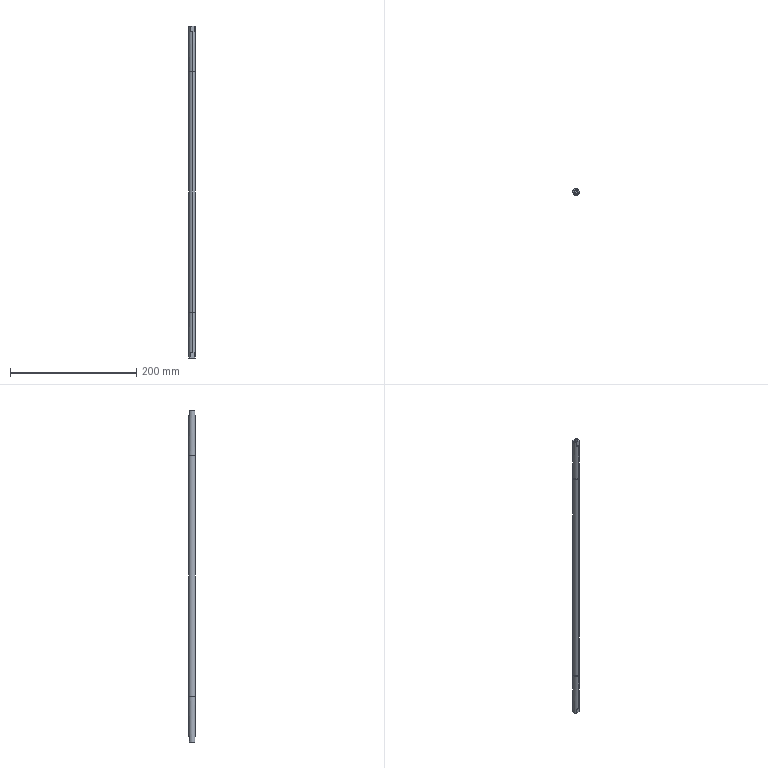Component | SolidWorks | Roller1-1-1_RollerAxis1-1 | 1 solid | 36 faces | box 10 x 10 x 525 mm | volume 40281 mm3 | cylinder 14 | plane 14 | cone 8 | commonest cylinder face diameters 10 x6 5 x4 9.65 x4
build123d program:
from build123d import *

# Parameters (mm, degrees)
CUT_EXTRUDE1_DEPTH           = 8
CUT_EXTRUDE2_DEPTH           = 8
CUT_EXTRUDE3_START           = -8
CUT_EXTRUDE3_DEPTH           = 8
CUT_EXTRUDE4_START           = -8
CUT_EXTRUDE4_DEPTH           = 8
F_5_0_5_DIAMETER_HOLE1_D     = 5
F_5_0_5_DIAMETER_HOLE1_DEPTH = 20
F_5_0_5_DIAMETER_HOLE1_TIP   = 1.502
F_5_0_5_DIAMETER_HOLE2_D     = 5
F_5_0_5_DIAMETER_HOLE2_DEPTH = 20
F_5_0_5_DIAMETER_HOLE2_TIP   = 1.502
CHAMFER1_SIZE                = 0.525


with BuildPart() as part:
    # Sketch1 → Revolve1 (revolve)
    with BuildSketch(Plane(origin=(0, 0, 0), x_dir=(-1, 0, 0), z_dir=(0, 0, -1)), mode=Mode.PRIVATE) as revolve1_sk:
        Polygon((-262.5, 5), (-262.5, 0), (262.5, 0), (262.5, 5), (191.1, 5), (191.1, 4.825), (190, 4.825), (190, 5), (-190, 5), (-190, 4.825), (-191.1, 4.825), (-191.1, 5), align=None)
    revolve(revolve1_sk.sketch.rotate(Axis((262.5, 0, 0), (-1, 0, 0)), 270), axis=Axis((262.5, 0, 0), (-1, 0, 0)))

    # Sketch2 → Cut-Extrude1 (cut)
    with BuildSketch(Plane(origin=(262.5, 0, 0), x_dir=(0, 0, -1), z_dir=(1, 0, 0))):
        with BuildLine():
            Line((4, 3), (4, -3))
            ThreePointArc((4, -3), (5, 0), (4, 3))
        make_face()
    extrude(amount=-CUT_EXTRUDE1_DEPTH, mode=Mode.SUBTRACT)

    # Sketch3 → Cut-Extrude2 (cut)
    with BuildSketch(Plane(origin=(262.5, 0, 0), x_dir=(0, 0, -1), z_dir=(1, 0, 0))):
        with BuildLine():
            Line((-4, -3), (-4, 3))
            ThreePointArc((-4, 3), (-5, 0), (-4, -3))
        make_face()
    extrude(amount=-CUT_EXTRUDE2_DEPTH, mode=Mode.SUBTRACT)

    # Sketch4 → Cut-Extrude3 (cut)
    with BuildSketch(Plane.ZY.offset(262.5).offset(CUT_EXTRUDE3_START)):
        with BuildLine():
            Line((-4, -3), (-4, 3))
            ThreePointArc((-4, 3), (-5, 0), (-4, -3))
        make_face()
    extrude(amount=CUT_EXTRUDE3_DEPTH, mode=Mode.SUBTRACT)

    # Sketch5 → Cut-Extrude4 (cut)
    with BuildSketch(Plane.ZY.offset(262.5).offset(CUT_EXTRUDE4_START)):
        with BuildLine():
            Line((4, 3), (4, -3))
            ThreePointArc((4, -3), (5, 0), (4, 3))
        make_face()
    extrude(amount=CUT_EXTRUDE4_DEPTH, mode=Mode.SUBTRACT)

    # 5.0 _5_ Diameter Hole1
    with Locations(Plane.ZY.offset(262.5)):
        with Locations((0, 0)):
            Hole(F_5_0_5_DIAMETER_HOLE1_D / 2, depth=F_5_0_5_DIAMETER_HOLE1_DEPTH)
            with Locations((0, 0, -(F_5_0_5_DIAMETER_HOLE1_DEPTH + F_5_0_5_DIAMETER_HOLE1_TIP / 2))):  # 118° drill point
                Cone(0, F_5_0_5_DIAMETER_HOLE1_D / 2, F_5_0_5_DIAMETER_HOLE1_TIP, mode=Mode.SUBTRACT)

    # 5.0 _5_ Diameter Hole2
    with Locations(Plane(origin=(262.5, 0, 0), x_dir=(0, 0, -1), z_dir=(1, 0, 0))):
        with Locations((0, 0)):
            Hole(F_5_0_5_DIAMETER_HOLE2_D / 2, depth=F_5_0_5_DIAMETER_HOLE2_DEPTH)
            with Locations((0, 0, -(F_5_0_5_DIAMETER_HOLE2_DEPTH + F_5_0_5_DIAMETER_HOLE2_TIP / 2))):  # 118° drill point
                Cone(0, F_5_0_5_DIAMETER_HOLE2_D / 2, F_5_0_5_DIAMETER_HOLE2_TIP, mode=Mode.SUBTRACT)

    # Chamfer1
    chamfer1_edges = [part.edges().sort_by_distance(p)[0] for p in [
        (-262.5, 0, 2.5),
        (262.5, 0, -2.5),
    ]]
    chamfer(chamfer1_edges, length=CHAMFER1_SIZE)


solid = part.part

# Placed as in the assembly
solid = solid.moved(Location((-44.993, 283.892, 0), (90, 5.533, 90)))
STEP:
#1=COLOUR_RGB('',0.7922,0.8196,0.9333);
#2=FILL_AREA_STYLE_COLOUR('',#1);
#3=FILL_AREA_STYLE('',(#2));
#4=SURFACE_STYLE_FILL_AREA(#3);
#5=SURFACE_SIDE_STYLE('',(#4));
#6=SURFACE_STYLE_USAGE(.BOTH.,#5);
#7=PRESENTATION_STYLE_ASSIGNMENT((#6));
#8=CARTESIAN_POINT('',(-1.762,11.079,-10.314));
#9=VERTEX_POINT('',#8);
#10=CARTESIAN_POINT('',(-1.781,11.275,-10.314));
#11=VERTEX_POINT('',#10);
#12=CARTESIAN_POINT('',(-1.771,11.177,-10.314));
#13=DIRECTION('',(-0.,0.,-1.));
#14=DIRECTION('',(-0.09642,0.9953,0.));
#15=AXIS2_PLACEMENT_3D('',#12,#13,#14);
#16=CIRCLE('',#15,0.09843);
#17=EDGE_CURVE('',#9,#11,#16,.T.);
#18=ORIENTED_EDGE('',*,*,#17,.F.);
#19=CARTESIAN_POINT('',(-1.76,11.058,-10.335));
#20=VERTEX_POINT('',#19);
#21=CARTESIAN_POINT('',(-1.762,11.079,-10.314));
#22=DIRECTION('',(0.06818,-0.7038,-0.7071));
#23=VECTOR('',#22,39.37);
#24=LINE('',#21,#23);
#25=EDGE_CURVE('',#9,#20,#24,.T.);
#26=ORIENTED_EDGE('',*,*,#25,.T.);
#27=CARTESIAN_POINT('',(-1.783,11.295,-10.335));
#28=VERTEX_POINT('',#27);
#29=CARTESIAN_POINT('',(-1.771,11.177,-10.335));
#30=DIRECTION('',(0.,-0.,1.));
#31=DIRECTION('',(-0.09642,0.9953,0.));
#32=AXIS2_PLACEMENT_3D('',#29,#30,#31);
#33=CIRCLE('',#32,0.1191);
#34=EDGE_CURVE('',#28,#20,#33,.T.);
#35=ORIENTED_EDGE('',*,*,#34,.F.);
#36=CARTESIAN_POINT('',(-1.781,11.275,-10.314));
#37=DIRECTION('',(-0.06818,0.7038,-0.7071));
#38=VECTOR('',#37,39.37);
#39=LINE('',#36,#38);
#40=EDGE_CURVE('',#11,#28,#39,.T.);
#41=ORIENTED_EDGE('',*,*,#40,.F.);
#42=EDGE_LOOP('',(#18,#26,#35,#41));
#43=FACE_OUTER_BOUND('',#42,.T.);
#44=CARTESIAN_POINT('',(-1.771,11.177,-10.314));
#45=DIRECTION('',(-0.,0.,-1.));
#46=DIRECTION('',(-0.09642,0.9953,0.));
#47=AXIS2_PLACEMENT_3D('',#44,#45,#46);
#48=CONICAL_SURFACE('',#47,0.09843,0.7854);
#49=ADVANCED_FACE('',(#43),#48,.F.);
#50=CARTESIAN_POINT('',(-1.781,11.275,10.314));
#51=VERTEX_POINT('',#50);
#52=CARTESIAN_POINT('',(-1.762,11.079,10.314));
#53=VERTEX_POINT('',#52);
#54=CARTESIAN_POINT('',(-1.771,11.177,10.314));
#55=DIRECTION('',(0.,-0.,1.));
#56=DIRECTION('',(0.09642,-0.9953,0.));
#57=AXIS2_PLACEMENT_3D('',#54,#55,#56);
#58=CIRCLE('',#57,0.09843);
#59=EDGE_CURVE('',#51,#53,#58,.T.);
#60=ORIENTED_EDGE('',*,*,#59,.F.);
#61=CARTESIAN_POINT('',(-1.783,11.295,10.335));
#62=VERTEX_POINT('',#61);
#63=CARTESIAN_POINT('',(-1.781,11.275,10.314));
#64=DIRECTION('',(-0.06818,0.7038,0.7071));
#65=VECTOR('',#64,39.37);
#66=LINE('',#63,#65);
#67=EDGE_CURVE('',#51,#62,#66,.T.);
#68=ORIENTED_EDGE('',*,*,#67,.T.);
#69=CARTESIAN_POINT('',(-1.76,11.058,10.335));
#70=VERTEX_POINT('',#69);
#71=CARTESIAN_POINT('',(-1.771,11.177,10.335));
#72=DIRECTION('',(-0.,0.,-1.));
#73=DIRECTION('',(0.09642,-0.9953,0.));
#74=AXIS2_PLACEMENT_3D('',#71,#72,#73);
#75=CIRCLE('',#74,0.1191);
#76=EDGE_CURVE('',#70,#62,#75,.T.);
#77=ORIENTED_EDGE('',*,*,#76,.F.);
#78=CARTESIAN_POINT('',(-1.762,11.079,10.314));
#79=DIRECTION('',(0.06818,-0.7038,0.7071));
#80=VECTOR('',#79,39.37);
#81=LINE('',#78,#80);
#82=EDGE_CURVE('',#53,#70,#81,.T.);
#83=ORIENTED_EDGE('',*,*,#82,.F.);
#84=EDGE_LOOP('',(#60,#68,#77,#83));
#85=FACE_OUTER_BOUND('',#84,.T.);
#86=CARTESIAN_POINT('',(-1.771,11.177,10.314));
#87=DIRECTION('',(0.,-0.,1.));
#88=DIRECTION('',(0.09642,-0.9953,0.));
#89=AXIS2_PLACEMENT_3D('',#86,#87,#88);
#90=CONICAL_SURFACE('',#89,0.09843,0.7854);
#91=ADVANCED_FACE('',(#85),#90,.F.);
#92=CARTESIAN_POINT('',(-1.762,11.079,-9.547));
#93=VERTEX_POINT('',#92);
#94=CARTESIAN_POINT('',(-1.781,11.275,-9.547));
#95=VERTEX_POINT('',#94);
#96=CARTESIAN_POINT('',(-1.771,11.177,-9.547));
#97=DIRECTION('',(-0.,0.,-1.));
#98=DIRECTION('',(-0.09642,0.9953,0.));
#99=AXIS2_PLACEMENT_3D('',#96,#97,#98);
#100=CIRCLE('',#99,0.09843);
#101=EDGE_CURVE('',#93,#95,#100,.T.);
#102=ORIENTED_EDGE('',*,*,#101,.F.);
#103=CARTESIAN_POINT('',(-1.762,11.079,-10.335));
#104=DIRECTION('',(-0.,0.,-1.));
#105=VECTOR('',#104,39.37);
#106=LINE('',#103,#105);
#107=EDGE_CURVE('',#93,#9,#106,.T.);
#108=ORIENTED_EDGE('',*,*,#107,.T.);
#109=ORIENTED_EDGE('',*,*,#17,.T.);
#110=CARTESIAN_POINT('',(-1.781,11.275,-10.335));
#111=DIRECTION('',(-0.,0.,-1.));
#112=VECTOR('',#111,39.37);
#113=LINE('',#110,#112);
#114=EDGE_CURVE('',#95,#11,#113,.T.);
#115=ORIENTED_EDGE('',*,*,#114,.F.);
#116=EDGE_LOOP('',(#102,#108,#109,#115));
#117=FACE_OUTER_BOUND('',#116,.T.);
#118=CARTESIAN_POINT('',(-1.771,11.177,-10.335));
#119=DIRECTION('',(-0.,0.,-1.));
#120=DIRECTION('',(-0.09642,0.9953,0.));
#121=AXIS2_PLACEMENT_3D('',#118,#119,#120);
#122=CYLINDRICAL_SURFACE('',#121,0.09843);
#123=ADVANCED_FACE('',(#117),#122,.F.);
#124=CARTESIAN_POINT('',(-1.771,11.177,-9.488));
#125=VERTEX_POINT('',#124);
#126=CARTESIAN_POINT('',(-1.781,11.275,-9.547));
#127=DIRECTION('',(-0.08265,0.8532,-0.515));
#128=VECTOR('',#127,39.37);
#129=LINE('',#126,#128);
#130=EDGE_CURVE('',#125,#95,#129,.T.);
#131=ORIENTED_EDGE('',*,*,#130,.F.);
#132=CARTESIAN_POINT('',(-1.762,11.079,-9.547));
#133=DIRECTION('',(0.08265,-0.8532,-0.515));
#134=VECTOR('',#133,39.37);
#135=LINE('',#132,#134);
#136=EDGE_CURVE('',#125,#93,#135,.T.);
#137=ORIENTED_EDGE('',*,*,#136,.T.);
#138=ORIENTED_EDGE('',*,*,#101,.T.);
#139=EDGE_LOOP('',(#131,#137,#138));
#140=FACE_OUTER_BOUND('',#139,.T.);
#141=CARTESIAN_POINT('',(-1.771,11.177,-9.547));
#142=DIRECTION('',(-0.,0.,-1.));
#143=DIRECTION('',(-0.09642,0.9953,0.));
#144=AXIS2_PLACEMENT_3D('',#141,#142,#143);
#145=CONICAL_SURFACE('',#144,0.09843,1.03);
#146=ADVANCED_FACE('',(#140),#145,.F.);
#147=CARTESIAN_POINT('',(-1.781,11.275,9.547));
#148=VERTEX_POINT('',#147);
#149=CARTESIAN_POINT('',(-1.762,11.079,9.547));
#150=VERTEX_POINT('',#149);
#151=CARTESIAN_POINT('',(-1.771,11.177,9.547));
#152=DIRECTION('',(0.,-0.,1.));
#153=DIRECTION('',(0.09642,-0.9953,0.));
#154=AXIS2_PLACEMENT_3D('',#151,#152,#153);
#155=CIRCLE('',#154,0.09843);
#156=EDGE_CURVE('',#148,#150,#155,.T.);
#157=ORIENTED_EDGE('',*,*,#156,.F.);
#158=CARTESIAN_POINT('',(-1.781,11.275,10.335));
#159=DIRECTION('',(0.,-0.,1.));
#160=VECTOR('',#159,39.37);
#161=LINE('',#158,#160);
#162=EDGE_CURVE('',#148,#51,#161,.T.);
#163=ORIENTED_EDGE('',*,*,#162,.T.);
#164=ORIENTED_EDGE('',*,*,#59,.T.);
#165=CARTESIAN_POINT('',(-1.762,11.079,10.335));
#166=DIRECTION('',(0.,-0.,1.));
#167=VECTOR('',#166,39.37);
#168=LINE('',#165,#167);
#169=EDGE_CURVE('',#150,#53,#168,.T.);
#170=ORIENTED_EDGE('',*,*,#169,.F.);
#171=EDGE_LOOP('',(#157,#163,#164,#170));
#172=FACE_OUTER_BOUND('',#171,.T.);
#173=CARTESIAN_POINT('',(-1.771,11.177,10.335));
#174=DIRECTION('',(0.,-0.,1.));
#175=DIRECTION('',(0.09642,-0.9953,0.));
#176=AXIS2_PLACEMENT_3D('',#173,#174,#175);
#177=CYLINDRICAL_SURFACE('',#176,0.09843);
#178=ADVANCED_FACE('',(#172),#177,.F.);
#179=CARTESIAN_POINT('',(-1.771,11.177,9.488));
#180=VERTEX_POINT('',#179);
#181=CARTESIAN_POINT('',(-1.762,11.079,9.547));
#182=DIRECTION('',(0.08265,-0.8532,0.515));
#183=VECTOR('',#182,39.37);
#184=LINE('',#181,#183);
#185=EDGE_CURVE('',#180,#150,#184,.T.);
#186=ORIENTED_EDGE('',*,*,#185,.F.);
#187=CARTESIAN_POINT('',(-1.781,11.275,9.547));
#188=DIRECTION('',(-0.08265,0.8532,0.515));
#189=VECTOR('',#188,39.37);
#190=LINE('',#187,#189);
#191=EDGE_CURVE('',#180,#148,#190,.T.);
#192=ORIENTED_EDGE('',*,*,#191,.T.);
#193=ORIENTED_EDGE('',*,*,#156,.T.);
#194=EDGE_LOOP('',(#186,#192,#193));
#195=FACE_OUTER_BOUND('',#194,.T.);
#196=CARTESIAN_POINT('',(-1.771,11.177,9.547));
#197=DIRECTION('',(0.,-0.,1.));
#198=DIRECTION('',(0.09642,-0.9953,0.));
#199=AXIS2_PLACEMENT_3D('',#196,#197,#198);
#200=CONICAL_SURFACE('',#199,0.09843,1.03);
#201=ADVANCED_FACE('',(#195),#200,.F.);
#202=CARTESIAN_POINT('',(-1.753,10.988,-7.524));
#203=VERTEX_POINT('',#202);
#204=CARTESIAN_POINT('',(-1.79,11.366,-7.524));
#205=VERTEX_POINT('',#204);
#206=CARTESIAN_POINT('',(-1.771,11.177,-7.524));
#207=DIRECTION('',(0.,-0.,1.));
#208=DIRECTION('',(0.09642,-0.9953,0.));
#209=AXIS2_PLACEMENT_3D('',#206,#207,#208);
#210=CIRCLE('',#209,0.19);
#211=EDGE_CURVE('',#203,#205,#210,.T.);
#212=ORIENTED_EDGE('',*,*,#211,.T.);
#213=CARTESIAN_POINT('',(-1.79,11.366,-7.48));
#214=VERTEX_POINT('',#213);
#215=CARTESIAN_POINT('',(-1.79,11.366,-10.335));
#216=DIRECTION('',(0.,-0.,1.));
#217=VECTOR('',#216,39.37);
#218=LINE('',#215,#217);
#219=EDGE_CURVE('',#205,#214,#218,.T.);
#220=ORIENTED_EDGE('',*,*,#219,.T.);
#221=CARTESIAN_POINT('',(-1.753,10.988,-7.48));
#222=VERTEX_POINT('',#221);
#223=CARTESIAN_POINT('',(-1.771,11.177,-7.48));
#224=DIRECTION('',(0.,-0.,1.));
#225=DIRECTION('',(0.09642,-0.9953,0.));
#226=AXIS2_PLACEMENT_3D('',#223,#224,#225);
#227=CIRCLE('',#226,0.19);
#228=EDGE_CURVE('',#222,#214,#227,.T.);
#229=ORIENTED_EDGE('',*,*,#228,.F.);
#230=CARTESIAN_POINT('',(-1.753,10.988,-10.335));
#231=DIRECTION('',(0.,-0.,1.));
#232=VECTOR('',#231,39.37);
#233=LINE('',#230,#232);
#234=EDGE_CURVE('',#203,#222,#233,.T.);
#235=ORIENTED_EDGE('',*,*,#234,.F.);
#236=EDGE_LOOP('',(#212,#220,#229,#235));
#237=FACE_OUTER_BOUND('',#236,.T.);
#238=CARTESIAN_POINT('',(-1.771,11.177,-10.335));
#239=DIRECTION('',(0.,-0.,1.));
#240=DIRECTION('',(0.09642,-0.9953,0.));
#241=AXIS2_PLACEMENT_3D('',#238,#239,#240);
#242=CYLINDRICAL_SURFACE('',#241,0.19);
#243=ADVANCED_FACE('',(#237),#242,.T.);
#244=CARTESIAN_POINT('',(-1.752,10.981,-7.48));
#245=VERTEX_POINT('',#244);
#246=CARTESIAN_POINT('',(-1.79,11.373,-7.48));
#247=VERTEX_POINT('',#246);
#248=CARTESIAN_POINT('',(-1.771,11.177,-7.48));
#249=DIRECTION('',(0.,-0.,1.));
#250=DIRECTION('',(0.09642,-0.9953,0.));
#251=AXIS2_PLACEMENT_3D('',#248,#249,#250);
#252=CIRCLE('',#251,0.1969);
#253=EDGE_CURVE('',#245,#247,#252,.T.);
#254=ORIENTED_EDGE('',*,*,#253,.T.);
#255=CARTESIAN_POINT('',(-1.79,11.373,7.48));
#256=VERTEX_POINT('',#255);
#257=CARTESIAN_POINT('',(-1.79,11.373,-10.335));
#258=DIRECTION('',(0.,-0.,1.));
#259=VECTOR('',#258,39.37);
#260=LINE('',#257,#259);
#261=EDGE_CURVE('',#247,#256,#260,.T.);
#262=ORIENTED_EDGE('',*,*,#261,.T.);
#263=CARTESIAN_POINT('',(-1.752,10.981,7.48));
#264=VERTEX_POINT('',#263);
#265=CARTESIAN_POINT('',(-1.771,11.177,7.48));
#266=DIRECTION('',(0.,-0.,1.));
#267=DIRECTION('',(0.09642,-0.9953,0.));
#268=AXIS2_PLACEMENT_3D('',#265,#266,#267);
#269=CIRCLE('',#268,0.1969);
#270=EDGE_CURVE('',#264,#256,#269,.T.);
#271=ORIENTED_EDGE('',*,*,#270,.F.);
#272=CARTESIAN_POINT('',(-1.752,10.981,-10.335));
#273=DIRECTION('',(0.,-0.,1.));
#274=VECTOR('',#273,39.37);
#275=LINE('',#272,#274);
#276=EDGE_CURVE('',#245,#264,#275,.T.);
#277=ORIENTED_EDGE('',*,*,#276,.F.);
#278=EDGE_LOOP('',(#254,#262,#271,#277));
#279=FACE_OUTER_BOUND('',#278,.T.);
#280=CARTESIAN_POINT('',(-1.771,11.177,-10.335));
#281=DIRECTION('',(0.,-0.,1.));
#282=DIRECTION('',(0.09642,-0.9953,0.));
#283=AXIS2_PLACEMENT_3D('',#280,#281,#282);
#284=CYLINDRICAL_SURFACE('',#283,0.1969);
#285=ADVANCED_FACE('',(#279),#284,.T.);
#286=CARTESIAN_POINT('',(-1.753,10.988,7.48));
#287=VERTEX_POINT('',#286);
#288=CARTESIAN_POINT('',(-1.79,11.366,7.48));
#289=VERTEX_POINT('',#288);
#290=CARTESIAN_POINT('',(-1.771,11.177,7.48));
#291=DIRECTION('',(0.,-0.,1.));
#292=DIRECTION('',(0.09642,-0.9953,0.));
#293=AXIS2_PLACEMENT_3D('',#290,#291,#292);
#294=CIRCLE('',#293,0.19);
#295=EDGE_CURVE('',#287,#289,#294,.T.);
#296=ORIENTED_EDGE('',*,*,#295,.T.);
#297=CARTESIAN_POINT('',(-1.79,11.366,7.524));
#298=VERTEX_POINT('',#297);
#299=CARTESIAN_POINT('',(-1.79,11.366,-10.335));
#300=DIRECTION('',(0.,-0.,1.));
#301=VECTOR('',#300,39.37);
#302=LINE('',#299,#301);
#303=EDGE_CURVE('',#289,#298,#302,.T.);
#304=ORIENTED_EDGE('',*,*,#303,.T.);
#305=CARTESIAN_POINT('',(-1.753,10.988,7.524));
#306=VERTEX_POINT('',#305);
#307=CARTESIAN_POINT('',(-1.771,11.177,7.524));
#308=DIRECTION('',(0.,-0.,1.));
#309=DIRECTION('',(0.09642,-0.9953,0.));
#310=AXIS2_PLACEMENT_3D('',#307,#308,#309);
#311=CIRCLE('',#310,0.19);
#312=EDGE_CURVE('',#306,#298,#311,.T.);
#313=ORIENTED_EDGE('',*,*,#312,.F.);
#314=CARTESIAN_POINT('',(-1.753,10.988,-10.335));
#315=DIRECTION('',(0.,-0.,1.));
#316=VECTOR('',#315,39.37);
#317=LINE('',#314,#316);
#318=EDGE_CURVE('',#287,#306,#317,.T.);
#319=ORIENTED_EDGE('',*,*,#318,.F.);
#320=EDGE_LOOP('',(#296,#304,#313,#319));
#321=FACE_OUTER_BOUND('',#320,.T.);
#322=CARTESIAN_POINT('',(-1.771,11.177,-10.335));
#323=DIRECTION('',(0.,-0.,1.));
#324=DIRECTION('',(0.09642,-0.9953,0.));
#325=AXIS2_PLACEMENT_3D('',#322,#323,#324);
#326=CYLINDRICAL_SURFACE('',#325,0.19);
#327=ADVANCED_FACE('',(#321),#326,.T.);
#328=CARTESIAN_POINT('',(-1.752,10.981,7.524));
#329=VERTEX_POINT('',#328);
#330=CARTESIAN_POINT('',(-1.79,11.373,7.524));
#331=VERTEX_POINT('',#330);
#332=CARTESIAN_POINT('',(-1.771,11.177,7.524));
#333=DIRECTION('',(0.,-0.,1.));
#334=DIRECTION('',(0.09642,-0.9953,0.));
#335=AXIS2_PLACEMENT_3D('',#332,#333,#334);
#336=CIRCLE('',#335,0.1969);
#337=EDGE_CURVE('',#329,#331,#336,.T.);
#338=ORIENTED_EDGE('',*,*,#337,.T.);
#339=CARTESIAN_POINT('',(-1.79,11.373,10.02));
#340=VERTEX_POINT('',#339);
#341=CARTESIAN_POINT('',(-1.79,11.373,-10.335));
#342=DIRECTION('',(0.,-0.,1.));
#343=VECTOR('',#342,39.37);
#344=LINE('',#341,#343);
#345=EDGE_CURVE('',#331,#340,#344,.T.);
#346=ORIENTED_EDGE('',*,*,#345,.T.);
#347=CARTESIAN_POINT('',(-1.669,11.345,10.02));
#348=VERTEX_POINT('',#347);
#349=CARTESIAN_POINT('',(-1.771,11.177,10.02));
#350=DIRECTION('',(0.,-0.,1.));
#351=DIRECTION('',(0.09642,-0.9953,0.));
#352=AXIS2_PLACEMENT_3D('',#349,#350,#351);
#353=CIRCLE('',#352,0.1969);
#354=EDGE_CURVE('',#348,#340,#353,.T.);
#355=ORIENTED_EDGE('',*,*,#354,.F.);
#356=CARTESIAN_POINT('',(-1.669,11.345,10.335));
#357=VERTEX_POINT('',#356);
#358=CARTESIAN_POINT('',(-1.669,11.345,10.02));
#359=DIRECTION('',(0.,-0.,1.));
#360=VECTOR('',#359,39.37);
#361=LINE('',#358,#360);
#362=EDGE_CURVE('',#348,#357,#361,.T.);
#363=ORIENTED_EDGE('',*,*,#362,.T.);
#364=CARTESIAN_POINT('',(-1.639,11.031,10.335));
#365=VERTEX_POINT('',#364);
#366=CARTESIAN_POINT('',(-1.771,11.177,10.335));
#367=DIRECTION('',(0.,-0.,1.));
#368=DIRECTION('',(0.09642,-0.9953,0.));
#369=AXIS2_PLACEMENT_3D('',#366,#367,#368);
#370=CIRCLE('',#369,0.1969);
#371=EDGE_CURVE('',#365,#357,#370,.T.);
#372=ORIENTED_EDGE('',*,*,#371,.F.);
#373=CARTESIAN_POINT('',(-1.639,11.031,10.02));
#374=VERTEX_POINT('',#373);
#375=CARTESIAN_POINT('',(-1.639,11.031,10.02));
#376=DIRECTION('',(0.,-0.,1.));
#377=VECTOR('',#376,39.37);
#378=LINE('',#375,#377);
#379=EDGE_CURVE('',#374,#365,#378,.T.);
#380=ORIENTED_EDGE('',*,*,#379,.F.);
#381=CARTESIAN_POINT('',(-1.752,10.981,10.02));
#382=VERTEX_POINT('',#381);
#383=CARTESIAN_POINT('',(-1.771,11.177,10.02));
#384=DIRECTION('',(0.,-0.,1.));
#385=DIRECTION('',(0.09642,-0.9953,0.));
#386=AXIS2_PLACEMENT_3D('',#383,#384,#385);
#387=CIRCLE('',#386,0.1969);
#388=EDGE_CURVE('',#382,#374,#387,.T.);
#389=ORIENTED_EDGE('',*,*,#388,.F.);
#390=CARTESIAN_POINT('',(-1.752,10.981,-10.335));
#391=DIRECTION('',(0.,-0.,1.));
#392=VECTOR('',#391,39.37);
#393=LINE('',#390,#392);
#394=EDGE_CURVE('',#329,#382,#393,.T.);
#395=ORIENTED_EDGE('',*,*,#394,.F.);
#396=EDGE_LOOP('',(#338,#346,#355,#363,#372,#380,#389,#395));
#397=FACE_OUTER_BOUND('',#396,.T.);
#398=CARTESIAN_POINT('',(-1.771,11.177,-10.335));
#399=DIRECTION('',(0.,-0.,1.));
#400=DIRECTION('',(0.09642,-0.9953,0.));
#401=AXIS2_PLACEMENT_3D('',#398,#399,#400);
#402=CYLINDRICAL_SURFACE('',#401,0.1969);
#403=ADVANCED_FACE('',(#397),#402,.T.);
#404=CARTESIAN_POINT('',(-1.79,11.373,-10.02));
#405=VERTEX_POINT('',#404);
#406=CARTESIAN_POINT('',(-1.669,11.345,-10.02));
#407=VERTEX_POINT('',#406);
#408=CARTESIAN_POINT('',(-1.771,11.177,-10.02));
#409=DIRECTION('',(-0.,0.,-1.));
#410=DIRECTION('',(-0.09642,0.9953,0.));
#411=AXIS2_PLACEMENT_3D('',#408,#409,#410);
#412=CIRCLE('',#411,0.1969);
#413=EDGE_CURVE('',#405,#407,#412,.T.);
#414=ORIENTED_EDGE('',*,*,#413,.F.);
#415=CARTESIAN_POINT('',(-1.79,11.373,-7.524));
#416=VERTEX_POINT('',#415);
#417=CARTESIAN_POINT('',(-1.79,11.373,-10.335));
#418=DIRECTION('',(0.,-0.,1.));
#419=VECTOR('',#418,39.37);
#420=LINE('',#417,#419);
#421=EDGE_CURVE('',#405,#416,#420,.T.);
#422=ORIENTED_EDGE('',*,*,#421,.T.);
#423=CARTESIAN_POINT('',(-1.752,10.981,-7.524));
#424=VERTEX_POINT('',#423);
#425=CARTESIAN_POINT('',(-1.771,11.177,-7.524));
#426=DIRECTION('',(0.,-0.,1.));
#427=DIRECTION('',(0.09642,-0.9953,0.));
#428=AXIS2_PLACEMENT_3D('',#425,#426,#427);
#429=CIRCLE('',#428,0.1969);
#430=EDGE_CURVE('',#424,#416,#429,.T.);
#431=ORIENTED_EDGE('',*,*,#430,.F.);
#432=CARTESIAN_POINT('',(-1.752,10.981,-10.02));
#433=VERTEX_POINT('',#432);
#434=CARTESIAN_POINT('',(-1.752,10.981,-10.335));
#435=DIRECTION('',(0.,-0.,1.));
#436=VECTOR('',#435,39.37);
#437=LINE('',#434,#436);
#438=EDGE_CURVE('',#433,#424,#437,.T.);
#439=ORIENTED_EDGE('',*,*,#438,.F.);
#440=CARTESIAN_POINT('',(-1.639,11.031,-10.02));
#441=VERTEX_POINT('',#440);
#442=CARTESIAN_POINT('',(-1.771,11.177,-10.02));
#443=DIRECTION('',(-0.,0.,-1.));
#444=DIRECTION('',(-0.09642,0.9953,0.));
#445=AXIS2_PLACEMENT_3D('',#442,#443,#444);
#446=CIRCLE('',#445,0.1969);
#447=EDGE_CURVE('',#441,#433,#446,.T.);
#448=ORIENTED_EDGE('',*,*,#447,.F.);
#449=CARTESIAN_POINT('',(-1.639,11.031,-10.335));
#450=VERTEX_POINT('',#449);
#451=CARTESIAN_POINT('',(-1.639,11.031,-10.02));
#452=DIRECTION('',(-0.,0.,-1.));
#453=VECTOR('',#452,39.37);
#454=LINE('',#451,#453);
#455=EDGE_CURVE('',#441,#450,#454,.T.);
#456=ORIENTED_EDGE('',*,*,#455,.T.);
#457=CARTESIAN_POINT('',(-1.669,11.345,-10.335));
#458=VERTEX_POINT('',#457);
#459=CARTESIAN_POINT('',(-1.771,11.177,-10.335));
#460=DIRECTION('',(0.,-0.,1.));
#461=DIRECTION('',(0.09642,-0.9953,0.));
#462=AXIS2_PLACEMENT_3D('',#459,#460,#461);
#463=CIRCLE('',#462,0.1969);
#464=EDGE_CURVE('',#450,#458,#463,.T.);
#465=ORIENTED_EDGE('',*,*,#464,.T.);
#466=CARTESIAN_POINT('',(-1.669,11.345,-10.02));
#467=DIRECTION('',(-0.,0.,-1.));
#468=VECTOR('',#467,39.37);
#469=LINE('',#466,#468);
#470=EDGE_CURVE('',#407,#458,#469,.T.);
#471=ORIENTED_EDGE('',*,*,#470,.F.);
#472=EDGE_LOOP('',(#414,#422,#431,#439,#448,#456,#465,#471));
#473=FACE_OUTER_BOUND('',#472,.T.);
#474=CARTESIAN_POINT('',(-1.771,11.177,-10.335));
#475=DIRECTION('',(0.,-0.,1.));
#476=DIRECTION('',(0.09642,-0.9953,0.));
#477=AXIS2_PLACEMENT_3D('',#474,#475,#476);
#478=CYLINDRICAL_SURFACE('',#477,0.1969);
#479=ADVANCED_FACE('',(#473),#478,.T.);
#480=ORIENTED_EDGE('',*,*,#421,.F.);
#481=CARTESIAN_POINT('',(-1.904,11.322,-10.02));
#482=VERTEX_POINT('',#481);
#483=CARTESIAN_POINT('',(-1.771,11.177,-10.02));
#484=DIRECTION('',(-0.,0.,-1.));
#485=DIRECTION('',(-0.09642,0.9953,0.));
#486=AXIS2_PLACEMENT_3D('',#483,#484,#485);
#487=CIRCLE('',#486,0.1969);
#488=EDGE_CURVE('',#482,#405,#487,.T.);
#489=ORIENTED_EDGE('',*,*,#488,.F.);
#490=CARTESIAN_POINT('',(-1.904,11.322,-10.335));
#491=VERTEX_POINT('',#490);
#492=CARTESIAN_POINT('',(-1.904,11.322,-10.02));
#493=DIRECTION('',(-0.,0.,-1.));
#494=VECTOR('',#493,39.37);
#495=LINE('',#492,#494);
#496=EDGE_CURVE('',#482,#491,#495,.T.);
#497=ORIENTED_EDGE('',*,*,#496,.T.);
#498=CARTESIAN_POINT('',(-1.874,11.009,-10.335));
#499=VERTEX_POINT('',#498);
#500=CARTESIAN_POINT('',(-1.771,11.177,-10.335));
#501=DIRECTION('',(0.,-0.,1.));
#502=DIRECTION('',(0.09642,-0.9953,0.));
#503=AXIS2_PLACEMENT_3D('',#500,#501,#502);
#504=CIRCLE('',#503,0.1969);
#505=EDGE_CURVE('',#491,#499,#504,.T.);
#506=ORIENTED_EDGE('',*,*,#505,.T.);
#507=CARTESIAN_POINT('',(-1.874,11.009,-10.02));
#508=VERTEX_POINT('',#507);
#509=CARTESIAN_POINT('',(-1.874,11.009,-10.02));
#510=DIRECTION('',(-0.,0.,-1.));
#511=VECTOR('',#510,39.37);
#512=LINE('',#509,#511);
#513=EDGE_CURVE('',#508,#499,#512,.T.);
#514=ORIENTED_EDGE('',*,*,#513,.F.);
#515=CARTESIAN_POINT('',(-1.771,11.177,-10.02));
#516=DIRECTION('',(-0.,0.,-1.));
#517=DIRECTION('',(-0.09642,0.9953,0.));
#518=AXIS2_PLACEMENT_3D('',#515,#516,#517);
#519=CIRCLE('',#518,0.1969);
#520=EDGE_CURVE('',#433,#508,#519,.T.);
#521=ORIENTED_EDGE('',*,*,#520,.F.);
#522=ORIENTED_EDGE('',*,*,#438,.T.);
#523=CARTESIAN_POINT('',(-1.771,11.177,-7.524));
#524=DIRECTION('',(0.,-0.,1.));
#525=DIRECTION('',(0.09642,-0.9953,0.));
#526=AXIS2_PLACEMENT_3D('',#523,#524,#525);
#527=CIRCLE('',#526,0.1969);
#528=EDGE_CURVE('',#416,#424,#527,.T.);
#529=ORIENTED_EDGE('',*,*,#528,.F.);
#530=EDGE_LOOP('',(#480,#489,#497,#506,#514,#521,#522,#529));
#531=FACE_OUTER_BOUND('',#530,.T.);
#532=CARTESIAN_POINT('',(-1.771,11.177,-10.335));
#533=DIRECTION('',(0.,-0.,1.));
#534=DIRECTION('',(0.09642,-0.9953,0.));
#535=AXIS2_PLACEMENT_3D('',#532,#533,#534);
#536=CYLINDRICAL_SURFACE('',#535,0.1969);
#537=ADVANCED_FACE('',(#531),#536,.T.);
#538=ORIENTED_EDGE('',*,*,#34,.T.);
#539=CARTESIAN_POINT('',(-1.771,11.177,-10.335));
#540=DIRECTION('',(0.,-0.,1.));
#541=DIRECTION('',(-0.09642,0.9953,0.));
#542=AXIS2_PLACEMENT_3D('',#539,#540,#541);
#543=CIRCLE('',#542,0.1191);
#544=EDGE_CURVE('',#20,#28,#543,.T.);
#545=ORIENTED_EDGE('',*,*,#544,.T.);
#546=EDGE_LOOP('',(#538,#545));
#547=FACE_BOUND('',#546,.T.);
#548=CARTESIAN_POINT('',(-1.874,11.009,-10.335));
#549=DIRECTION('',(0.9953,0.09642,-0.));
#550=VECTOR('',#549,39.37);
#551=LINE('',#548,#550);
#552=EDGE_CURVE('',#499,#450,#551,.T.);
#553=ORIENTED_EDGE('',*,*,#552,.F.);
#554=ORIENTED_EDGE('',*,*,#505,.F.);
#555=CARTESIAN_POINT('',(-1.669,11.345,-10.335));
#556=DIRECTION('',(-0.9953,-0.09642,0.));
#557=VECTOR('',#556,39.37);
#558=LINE('',#555,#557);
#559=EDGE_CURVE('',#458,#491,#558,.T.);
#560=ORIENTED_EDGE('',*,*,#559,.F.);
#561=ORIENTED_EDGE('',*,*,#464,.F.);
#562=EDGE_LOOP('',(#553,#554,#560,#561));
#563=FACE_OUTER_BOUND('',#562,.T.);
#564=CARTESIAN_POINT('',(-1.575,11.196,-10.335));
#565=DIRECTION('',(-0.,0.,-1.));
#566=DIRECTION('',(-0.09642,0.9953,0.));
#567=AXIS2_PLACEMENT_3D('',#564,#565,#566);
#568=PLANE('',#567);
#569=ADVANCED_FACE('',(#547,#563),#568,.T.);
#570=ORIENTED_EDGE('',*,*,#76,.T.);
#571=CARTESIAN_POINT('',(-1.771,11.177,10.335));
#572=DIRECTION('',(-0.,0.,-1.));
#573=DIRECTION('',(0.09642,-0.9953,0.));
#574=AXIS2_PLACEMENT_3D('',#571,#572,#573);
#575=CIRCLE('',#574,0.1191);
#576=EDGE_CURVE('',#62,#70,#575,.T.);
#577=ORIENTED_EDGE('',*,*,#576,.T.);
#578=EDGE_LOOP('',(#570,#577));
#579=FACE_BOUND('',#578,.T.);
#580=CARTESIAN_POINT('',(-1.874,11.009,10.335));
#581=VERTEX_POINT('',#580);
#582=CARTESIAN_POINT('',(-1.639,11.031,10.335));
#583=DIRECTION('',(-0.9953,-0.09642,0.));
#584=VECTOR('',#583,39.37);
#585=LINE('',#582,#584);
#586=EDGE_CURVE('',#365,#581,#585,.T.);
#587=ORIENTED_EDGE('',*,*,#586,.F.);
#588=ORIENTED_EDGE('',*,*,#371,.T.);
#589=CARTESIAN_POINT('',(-1.904,11.322,10.335));
#590=VERTEX_POINT('',#589);
#591=CARTESIAN_POINT('',(-1.904,11.322,10.335));
#592=DIRECTION('',(0.9953,0.09642,-0.));
#593=VECTOR('',#592,39.37);
#594=LINE('',#591,#593);
#595=EDGE_CURVE('',#590,#357,#594,.T.);
#596=ORIENTED_EDGE('',*,*,#595,.F.);
#597=CARTESIAN_POINT('',(-1.771,11.177,10.335));
#598=DIRECTION('',(0.,-0.,1.));
#599=DIRECTION('',(0.09642,-0.9953,0.));
#600=AXIS2_PLACEMENT_3D('',#597,#598,#599);
#601=CIRCLE('',#600,0.1969);
#602=EDGE_CURVE('',#590,#581,#601,.T.);
#603=ORIENTED_EDGE('',*,*,#602,.T.);
#604=EDGE_LOOP('',(#587,#588,#596,#603));
#605=FACE_OUTER_BOUND('',#604,.T.);
#606=CARTESIAN_POINT('',(-1.771,11.177,10.335));
#607=DIRECTION('',(0.,-0.,1.));
#608=DIRECTION('',(0.09642,-0.9953,-0.));
#609=AXIS2_PLACEMENT_3D('',#606,#607,#608);
#610=PLANE('',#609);
#611=ADVANCED_FACE('',(#579,#605),#610,.T.);
#612=ORIENTED_EDGE('',*,*,#345,.F.);
#613=CARTESIAN_POINT('',(-1.771,11.177,7.524));
#614=DIRECTION('',(0.,-0.,1.));
#615=DIRECTION('',(0.09642,-0.9953,0.));
#616=AXIS2_PLACEMENT_3D('',#613,#614,#615);
#617=CIRCLE('',#616,0.1969);
#618=EDGE_CURVE('',#331,#329,#617,.T.);
#619=ORIENTED_EDGE('',*,*,#618,.T.);
#620=ORIENTED_EDGE('',*,*,#394,.T.);
#621=CARTESIAN_POINT('',(-1.874,11.009,10.02));
#622=VERTEX_POINT('',#621);
#623=CARTESIAN_POINT('',(-1.771,11.177,10.02));
#624=DIRECTION('',(0.,-0.,1.));
#625=DIRECTION('',(0.09642,-0.9953,0.));
#626=AXIS2_PLACEMENT_3D('',#623,#624,#625);
#627=CIRCLE('',#626,0.1969);
#628=EDGE_CURVE('',#622,#382,#627,.T.);
#629=ORIENTED_EDGE('',*,*,#628,.F.);
#630=CARTESIAN_POINT('',(-1.874,11.009,10.02));
#631=DIRECTION('',(0.,-0.,1.));
#632=VECTOR('',#631,39.37);
#633=LINE('',#630,#632);
#634=EDGE_CURVE('',#622,#581,#633,.T.);
#635=ORIENTED_EDGE('',*,*,#634,.T.);
#636=ORIENTED_EDGE('',*,*,#602,.F.);
#637=CARTESIAN_POINT('',(-1.904,11.322,10.02));
#638=VERTEX_POINT('',#637);
#639=CARTESIAN_POINT('',(-1.904,11.322,10.02));
#640=DIRECTION('',(0.,-0.,1.));
#641=VECTOR('',#640,39.37);
#642=LINE('',#639,#641);
#643=EDGE_CURVE('',#638,#590,#642,.T.);
#644=ORIENTED_EDGE('',*,*,#643,.F.);
#645=CARTESIAN_POINT('',(-1.771,11.177,10.02));
#646=DIRECTION('',(0.,-0.,1.));
#647=DIRECTION('',(0.09642,-0.9953,0.));
#648=AXIS2_PLACEMENT_3D('',#645,#646,#647);
#649=CIRCLE('',#648,0.1969);
#650=EDGE_CURVE('',#340,#638,#649,.T.);
#651=ORIENTED_EDGE('',*,*,#650,.F.);
#652=EDGE_LOOP('',(#612,#619,#620,#629,#635,#636,#644,#651));
#653=FACE_OUTER_BOUND('',#652,.T.);
#654=CARTESIAN_POINT('',(-1.771,11.177,-10.335));
#655=DIRECTION('',(0.,-0.,1.));
#656=DIRECTION('',(0.09642,-0.9953,0.));
#657=AXIS2_PLACEMENT_3D('',#654,#655,#656);
#658=CYLINDRICAL_SURFACE('',#657,0.1969);
#659=ADVANCED_FACE('',(#653),#658,.T.);
#660=ORIENTED_EDGE('',*,*,#312,.T.);
#661=CARTESIAN_POINT('',(-1.771,11.177,7.524));
#662=DIRECTION('',(0.,-0.,1.));
#663=DIRECTION('',(0.09642,-0.9953,0.));
#664=AXIS2_PLACEMENT_3D('',#661,#662,#663);
#665=CIRCLE('',#664,0.19);
#666=EDGE_CURVE('',#298,#306,#665,.T.);
#667=ORIENTED_EDGE('',*,*,#666,.T.);
#668=EDGE_LOOP('',(#660,#667));
#669=FACE_BOUND('',#668,.T.);
#670=ORIENTED_EDGE('',*,*,#337,.F.);
#671=ORIENTED_EDGE('',*,*,#618,.F.);
#672=EDGE_LOOP('',(#670,#671));
#673=FACE_OUTER_BOUND('',#672,.T.);
#674=CARTESIAN_POINT('',(-1.575,11.196,7.524));
#675=DIRECTION('',(-0.,0.,-1.));
#676=DIRECTION('',(-0.09642,0.9953,0.));
#677=AXIS2_PLACEMENT_3D('',#674,#675,#676);
#678=PLANE('',#677);
#679=ADVANCED_FACE('',(#669,#673),#678,.T.);
#680=ORIENTED_EDGE('',*,*,#303,.F.);
#681=CARTESIAN_POINT('',(-1.771,11.177,7.48));
#682=DIRECTION('',(0.,-0.,1.));
#683=DIRECTION('',(0.09642,-0.9953,0.));
#684=AXIS2_PLACEMENT_3D('',#681,#682,#683);
#685=CIRCLE('',#684,0.19);
#686=EDGE_CURVE('',#289,#287,#685,.T.);
#687=ORIENTED_EDGE('',*,*,#686,.T.);
#688=ORIENTED_EDGE('',*,*,#318,.T.);
#689=ORIENTED_EDGE('',*,*,#666,.F.);
#690=EDGE_LOOP('',(#680,#687,#688,#689));
#691=FACE_OUTER_BOUND('',#690,.T.);
#692=CARTESIAN_POINT('',(-1.771,11.177,-10.335));
#693=DIRECTION('',(0.,-0.,1.));
#694=DIRECTION('',(0.09642,-0.9953,0.));
#695=AXIS2_PLACEMENT_3D('',#692,#693,#694);
#696=CYLINDRICAL_SURFACE('',#695,0.19);
#697=ADVANCED_FACE('',(#691),#696,.T.);
#698=ORIENTED_EDGE('',*,*,#270,.T.);
#699=CARTESIAN_POINT('',(-1.771,11.177,7.48));
#700=DIRECTION('',(0.,-0.,1.));
#701=DIRECTION('',(0.09642,-0.9953,0.));
#702=AXIS2_PLACEMENT_3D('',#699,#700,#701);
#703=CIRCLE('',#702,0.1969);
#704=EDGE_CURVE('',#256,#264,#703,.T.);
#705=ORIENTED_EDGE('',*,*,#704,.T.);
#706=EDGE_LOOP('',(#698,#705));
#707=FACE_OUTER_BOUND('',#706,.T.);
#708=ORIENTED_EDGE('',*,*,#295,.F.);
#709=ORIENTED_EDGE('',*,*,#686,.F.);
#710=EDGE_LOOP('',(#708,#709));
#711=FACE_BOUND('',#710,.T.);
#712=CARTESIAN_POINT('',(-1.582,11.195,7.48));
#713=DIRECTION('',(0.,-0.,1.));
#714=DIRECTION('',(0.09642,-0.9953,-0.));
#715=AXIS2_PLACEMENT_3D('',#712,#713,#714);
#716=PLANE('',#715);
#717=ADVANCED_FACE('',(#707,#711),#716,.T.);
#718=ORIENTED_EDGE('',*,*,#261,.F.);
#719=CARTESIAN_POINT('',(-1.771,11.177,-7.48));
#720=DIRECTION('',(0.,-0.,1.));
#721=DIRECTION('',(0.09642,-0.9953,0.));
#722=AXIS2_PLACEMENT_3D('',#719,#720,#721);
#723=CIRCLE('',#722,0.1969);
#724=EDGE_CURVE('',#247,#245,#723,.T.);
#725=ORIENTED_EDGE('',*,*,#724,.T.);
#726=ORIENTED_EDGE('',*,*,#276,.T.);
#727=ORIENTED_EDGE('',*,*,#704,.F.);
#728=EDGE_LOOP('',(#718,#725,#726,#727));
#729=FACE_OUTER_BOUND('',#728,.T.);
#730=CARTESIAN_POINT('',(-1.771,11.177,-10.335));
#731=DIRECTION('',(0.,-0.,1.));
#732=DIRECTION('',(0.09642,-0.9953,0.));
#733=AXIS2_PLACEMENT_3D('',#730,#731,#732);
#734=CYLINDRICAL_SURFACE('',#733,0.1969);
#735=ADVANCED_FACE('',(#729),#734,.T.);
#736=ORIENTED_EDGE('',*,*,#228,.T.);
#737=CARTESIAN_POINT('',(-1.771,11.177,-7.48));
#738=DIRECTION('',(0.,-0.,1.));
#739=DIRECTION('',(0.09642,-0.9953,0.));
#740=AXIS2_PLACEMENT_3D('',#737,#738,#739);
#741=CIRCLE('',#740,0.19);
#742=EDGE_CURVE('',#214,#222,#741,.T.);
#743=ORIENTED_EDGE('',*,*,#742,.T.);
#744=EDGE_LOOP('',(#736,#743));
#745=FACE_BOUND('',#744,.T.);
#746=ORIENTED_EDGE('',*,*,#253,.F.);
#747=ORIENTED_EDGE('',*,*,#724,.F.);
#748=EDGE_LOOP('',(#746,#747));
#749=FACE_OUTER_BOUND('',#748,.T.);
#750=CARTESIAN_POINT('',(-1.575,11.196,-7.48));
#751=DIRECTION('',(-0.,0.,-1.));
#752=DIRECTION('',(-0.09642,0.9953,0.));
#753=AXIS2_PLACEMENT_3D('',#750,#751,#752);
#754=PLANE('',#753);
#755=ADVANCED_FACE('',(#745,#749),#754,.T.);
#756=ORIENTED_EDGE('',*,*,#219,.F.);
#757=CARTESIAN_POINT('',(-1.771,11.177,-7.524));
#758=DIRECTION('',(0.,-0.,1.));
#759=DIRECTION('',(0.09642,-0.9953,0.));
#760=AXIS2_PLACEMENT_3D('',#757,#758,#759);
#761=CIRCLE('',#760,0.19);
#762=EDGE_CURVE('',#205,#203,#761,.T.);
#763=ORIENTED_EDGE('',*,*,#762,.T.);
#764=ORIENTED_EDGE('',*,*,#234,.T.);
#765=ORIENTED_EDGE('',*,*,#742,.F.);
#766=EDGE_LOOP('',(#756,#763,#764,#765));
#767=FACE_OUTER_BOUND('',#766,.T.);
#768=CARTESIAN_POINT('',(-1.771,11.177,-10.335));
#769=DIRECTION('',(0.,-0.,1.));
#770=DIRECTION('',(0.09642,-0.9953,0.));
#771=AXIS2_PLACEMENT_3D('',#768,#769,#770);
#772=CYLINDRICAL_SURFACE('',#771,0.19);
#773=ADVANCED_FACE('',(#767),#772,.T.);
#774=ORIENTED_EDGE('',*,*,#430,.T.);
#775=ORIENTED_EDGE('',*,*,#528,.T.);
#776=EDGE_LOOP('',(#774,#775));
#777=FACE_OUTER_BOUND('',#776,.T.);
#778=ORIENTED_EDGE('',*,*,#211,.F.);
#779=ORIENTED_EDGE('',*,*,#762,.F.);
#780=EDGE_LOOP('',(#778,#779));
#781=FACE_BOUND('',#780,.T.);
#782=CARTESIAN_POINT('',(-1.582,11.195,-7.524));
#783=DIRECTION('',(0.,-0.,1.));
#784=DIRECTION('',(0.09642,-0.9953,-0.));
#785=AXIS2_PLACEMENT_3D('',#782,#783,#784);
#786=PLANE('',#785);
#787=ADVANCED_FACE('',(#777,#781),#786,.T.);
#788=ORIENTED_EDGE('',*,*,#559,.T.);
#789=ORIENTED_EDGE('',*,*,#496,.F.);
#790=CARTESIAN_POINT('',(-1.669,11.345,-10.02));
#791=DIRECTION('',(-0.9953,-0.09642,0.));
#792=VECTOR('',#791,39.37);
#793=LINE('',#790,#792);
#794=EDGE_CURVE('',#407,#482,#793,.T.);
#795=ORIENTED_EDGE('',*,*,#794,.F.);
#796=ORIENTED_EDGE('',*,*,#470,.T.);
#797=EDGE_LOOP('',(#788,#789,#795,#796));
#798=FACE_OUTER_BOUND('',#797,.T.);
#799=CARTESIAN_POINT('',(-1.669,11.345,-10.02));
#800=DIRECTION('',(0.09642,-0.9953,-0.));
#801=DIRECTION('',(-0.9953,-0.09642,0.));
#802=AXIS2_PLACEMENT_3D('',#799,#800,#801);
#803=PLANE('',#802);
#804=ADVANCED_FACE('',(#798),#803,.F.);
#805=ORIENTED_EDGE('',*,*,#488,.T.);
#806=ORIENTED_EDGE('',*,*,#413,.T.);
#807=ORIENTED_EDGE('',*,*,#794,.T.);
#808=EDGE_LOOP('',(#805,#806,#807));
#809=FACE_OUTER_BOUND('',#808,.T.);
#810=CARTESIAN_POINT('',(-1.771,11.177,-10.02));
#811=DIRECTION('',(-0.,0.,-1.));
#812=DIRECTION('',(-0.09642,0.9953,0.));
#813=AXIS2_PLACEMENT_3D('',#810,#811,#812);
#814=PLANE('',#813);
#815=ADVANCED_FACE('',(#809),#814,.T.);
#816=ORIENTED_EDGE('',*,*,#552,.T.);
#817=ORIENTED_EDGE('',*,*,#455,.F.);
#818=CARTESIAN_POINT('',(-1.874,11.009,-10.02));
#819=DIRECTION('',(0.9953,0.09642,-0.));
#820=VECTOR('',#819,39.37);
#821=LINE('',#818,#820);
#822=EDGE_CURVE('',#508,#441,#821,.T.);
#823=ORIENTED_EDGE('',*,*,#822,.F.);
#824=ORIENTED_EDGE('',*,*,#513,.T.);
#825=EDGE_LOOP('',(#816,#817,#823,#824));
#826=FACE_OUTER_BOUND('',#825,.T.);
#827=CARTESIAN_POINT('',(-1.874,11.009,-10.02));
#828=DIRECTION('',(-0.09642,0.9953,0.));
#829=DIRECTION('',(0.9953,0.09642,-0.));
#830=AXIS2_PLACEMENT_3D('',#827,#828,#829);
#831=PLANE('',#830);
#832=ADVANCED_FACE('',(#826),#831,.F.);
#833=ORIENTED_EDGE('',*,*,#447,.T.);
#834=ORIENTED_EDGE('',*,*,#520,.T.);
#835=ORIENTED_EDGE('',*,*,#822,.T.);
#836=EDGE_LOOP('',(#833,#834,#835));
#837=FACE_OUTER_BOUND('',#836,.T.);
#838=CARTESIAN_POINT('',(-1.771,11.177,-10.02));
#839=DIRECTION('',(-0.,0.,-1.));
#840=DIRECTION('',(-0.09642,0.9953,0.));
#841=AXIS2_PLACEMENT_3D('',#838,#839,#840);
#842=PLANE('',#841);
#843=ADVANCED_FACE('',(#837),#842,.T.);
#844=ORIENTED_EDGE('',*,*,#595,.T.);
#845=ORIENTED_EDGE('',*,*,#362,.F.);
#846=CARTESIAN_POINT('',(-1.904,11.322,10.02));
#847=DIRECTION('',(0.9953,0.09642,-0.));
#848=VECTOR('',#847,39.37);
#849=LINE('',#846,#848);
#850=EDGE_CURVE('',#638,#348,#849,.T.);
#851=ORIENTED_EDGE('',*,*,#850,.F.);
#852=ORIENTED_EDGE('',*,*,#643,.T.);
#853=EDGE_LOOP('',(#844,#845,#851,#852));
#854=FACE_OUTER_BOUND('',#853,.T.);
#855=CARTESIAN_POINT('',(-1.904,11.322,10.02));
#856=DIRECTION('',(0.09642,-0.9953,-0.));
#857=DIRECTION('',(-0.9953,-0.09642,0.));
#858=AXIS2_PLACEMENT_3D('',#855,#856,#857);
#859=PLANE('',#858);
#860=ADVANCED_FACE('',(#854),#859,.F.);
#861=ORIENTED_EDGE('',*,*,#354,.T.);
#862=ORIENTED_EDGE('',*,*,#650,.T.);
#863=ORIENTED_EDGE('',*,*,#850,.T.);
#864=EDGE_LOOP('',(#861,#862,#863));
#865=FACE_OUTER_BOUND('',#864,.T.);
#866=CARTESIAN_POINT('',(-1.771,11.177,10.02));
#867=DIRECTION('',(0.,-0.,1.));
#868=DIRECTION('',(0.09642,-0.9953,-0.));
#869=AXIS2_PLACEMENT_3D('',#866,#867,#868);
#870=PLANE('',#869);
#871=ADVANCED_FACE('',(#865),#870,.T.);
#872=ORIENTED_EDGE('',*,*,#586,.T.);
#873=ORIENTED_EDGE('',*,*,#634,.F.);
#874=CARTESIAN_POINT('',(-1.639,11.031,10.02));
#875=DIRECTION('',(-0.9953,-0.09642,0.));
#876=VECTOR('',#875,39.37);
#877=LINE('',#874,#876);
#878=EDGE_CURVE('',#374,#622,#877,.T.);
#879=ORIENTED_EDGE('',*,*,#878,.F.);
#880=ORIENTED_EDGE('',*,*,#379,.T.);
#881=EDGE_LOOP('',(#872,#873,#879,#880));
#882=FACE_OUTER_BOUND('',#881,.T.);
#883=CARTESIAN_POINT('',(-1.639,11.031,10.02));
#884=DIRECTION('',(-0.09642,0.9953,0.));
#885=DIRECTION('',(0.9953,0.09642,-0.));
#886=AXIS2_PLACEMENT_3D('',#883,#884,#885);
#887=PLANE('',#886);
#888=ADVANCED_FACE('',(#882),#887,.F.);
#889=ORIENTED_EDGE('',*,*,#628,.T.);
#890=ORIENTED_EDGE('',*,*,#388,.T.);
#891=ORIENTED_EDGE('',*,*,#878,.T.);
#892=EDGE_LOOP('',(#889,#890,#891));
#893=FACE_OUTER_BOUND('',#892,.T.);
#894=CARTESIAN_POINT('',(-1.771,11.177,10.02));
#895=DIRECTION('',(0.,-0.,1.));
#896=DIRECTION('',(0.09642,-0.9953,-0.));
#897=AXIS2_PLACEMENT_3D('',#894,#895,#896);
#898=PLANE('',#897);
#899=ADVANCED_FACE('',(#893),#898,.T.);
#900=ORIENTED_EDGE('',*,*,#191,.F.);
#901=ORIENTED_EDGE('',*,*,#185,.T.);
#902=CARTESIAN_POINT('',(-1.771,11.177,9.547));
#903=DIRECTION('',(0.,-0.,1.));
#904=DIRECTION('',(0.09642,-0.9953,0.));
#905=AXIS2_PLACEMENT_3D('',#902,#903,#904);
#906=CIRCLE('',#905,0.09843);
#907=EDGE_CURVE('',#150,#148,#906,.T.);
#908=ORIENTED_EDGE('',*,*,#907,.T.);
#909=EDGE_LOOP('',(#900,#901,#908));
#910=FACE_OUTER_BOUND('',#909,.T.);
#911=CARTESIAN_POINT('',(-1.771,11.177,9.547));
#912=DIRECTION('',(0.,-0.,1.));
#913=DIRECTION('',(0.09642,-0.9953,0.));
#914=AXIS2_PLACEMENT_3D('',#911,#912,#913);
#915=CONICAL_SURFACE('',#914,0.09843,1.03);
#916=ADVANCED_FACE('',(#910),#915,.F.);
#917=ORIENTED_EDGE('',*,*,#162,.F.);
#918=ORIENTED_EDGE('',*,*,#907,.F.);
#919=ORIENTED_EDGE('',*,*,#169,.T.);
#920=CARTESIAN_POINT('',(-1.771,11.177,10.314));
#921=DIRECTION('',(0.,-0.,1.));
#922=DIRECTION('',(0.09642,-0.9953,0.));
#923=AXIS2_PLACEMENT_3D('',#920,#921,#922);
#924=CIRCLE('',#923,0.09843);
#925=EDGE_CURVE('',#53,#51,#924,.T.);
#926=ORIENTED_EDGE('',*,*,#925,.T.);
#927=EDGE_LOOP('',(#917,#918,#919,#926));
#928=FACE_OUTER_BOUND('',#927,.T.);
#929=CARTESIAN_POINT('',(-1.771,11.177,10.335));
#930=DIRECTION('',(0.,-0.,1.));
#931=DIRECTION('',(0.09642,-0.9953,0.));
#932=AXIS2_PLACEMENT_3D('',#929,#930,#931);
#933=CYLINDRICAL_SURFACE('',#932,0.09843);
#934=ADVANCED_FACE('',(#928),#933,.F.);
#935=ORIENTED_EDGE('',*,*,#136,.F.);
#936=ORIENTED_EDGE('',*,*,#130,.T.);
#937=CARTESIAN_POINT('',(-1.771,11.177,-9.547));
#938=DIRECTION('',(-0.,0.,-1.));
#939=DIRECTION('',(-0.09642,0.9953,0.));
#940=AXIS2_PLACEMENT_3D('',#937,#938,#939);
#941=CIRCLE('',#940,0.09843);
#942=EDGE_CURVE('',#95,#93,#941,.T.);
#943=ORIENTED_EDGE('',*,*,#942,.T.);
#944=EDGE_LOOP('',(#935,#936,#943));
#945=FACE_OUTER_BOUND('',#944,.T.);
#946=CARTESIAN_POINT('',(-1.771,11.177,-9.547));
#947=DIRECTION('',(-0.,0.,-1.));
#948=DIRECTION('',(-0.09642,0.9953,0.));
#949=AXIS2_PLACEMENT_3D('',#946,#947,#948);
#950=CONICAL_SURFACE('',#949,0.09843,1.03);
#951=ADVANCED_FACE('',(#945),#950,.F.);
#952=ORIENTED_EDGE('',*,*,#107,.F.);
#953=ORIENTED_EDGE('',*,*,#942,.F.);
#954=ORIENTED_EDGE('',*,*,#114,.T.);
#955=CARTESIAN_POINT('',(-1.771,11.177,-10.314));
#956=DIRECTION('',(-0.,0.,-1.));
#957=DIRECTION('',(-0.09642,0.9953,0.));
#958=AXIS2_PLACEMENT_3D('',#955,#956,#957);
#959=CIRCLE('',#958,0.09843);
#960=EDGE_CURVE('',#11,#9,#959,.T.);
#961=ORIENTED_EDGE('',*,*,#960,.T.);
#962=EDGE_LOOP('',(#952,#953,#954,#961));
#963=FACE_OUTER_BOUND('',#962,.T.);
#964=CARTESIAN_POINT('',(-1.771,11.177,-10.335));
#965=DIRECTION('',(-0.,0.,-1.));
#966=DIRECTION('',(-0.09642,0.9953,0.));
#967=AXIS2_PLACEMENT_3D('',#964,#965,#966);
#968=CYLINDRICAL_SURFACE('',#967,0.09843);
#969=ADVANCED_FACE('',(#963),#968,.F.);
#970=ORIENTED_EDGE('',*,*,#67,.F.);
#971=ORIENTED_EDGE('',*,*,#925,.F.);
#972=ORIENTED_EDGE('',*,*,#82,.T.);
#973=ORIENTED_EDGE('',*,*,#576,.F.);
#974=EDGE_LOOP('',(#970,#971,#972,#973));
#975=FACE_OUTER_BOUND('',#974,.T.);
#976=CARTESIAN_POINT('',(-1.771,11.177,10.314));
#977=DIRECTION('',(0.,-0.,1.));
#978=DIRECTION('',(0.09642,-0.9953,0.));
#979=AXIS2_PLACEMENT_3D('',#976,#977,#978);
#980=CONICAL_SURFACE('',#979,0.09843,0.7854);
#981=ADVANCED_FACE('',(#975),#980,.F.);
#982=ORIENTED_EDGE('',*,*,#25,.F.);
#983=ORIENTED_EDGE('',*,*,#960,.F.);
#984=ORIENTED_EDGE('',*,*,#40,.T.);
#985=ORIENTED_EDGE('',*,*,#544,.F.);
#986=EDGE_LOOP('',(#982,#983,#984,#985));
#987=FACE_OUTER_BOUND('',#986,.T.);
#988=CARTESIAN_POINT('',(-1.771,11.177,-10.314));
#989=DIRECTION('',(-0.,0.,-1.));
#990=DIRECTION('',(-0.09642,0.9953,0.));
#991=AXIS2_PLACEMENT_3D('',#988,#989,#990);
#992=CONICAL_SURFACE('',#991,0.09843,0.7854);
#993=ADVANCED_FACE('',(#987),#992,.F.);
#994=CLOSED_SHELL('',(#49,#91,#123,#146,#178,#201,#243,#285,#327,#403,#479,#537,#569,#611,#659,#679,#697,#717,#735,#755,#773,#787,#804,#815,#832,#843,#860,#871,#888,#899,#916,#934,#951,#969,#981,#993));
#995=MANIFOLD_SOLID_BREP('',#994);
#996=STYLED_ITEM('',(#7),#995);
#997=PRESENTATION_LAYER_ASSIGNMENT('','',(#996));
#998=CARTESIAN_POINT('',(0.,0.,0.));
#999=DIRECTION('',(0.,0.,1.));
#1000=DIRECTION('',(1.,0.,0.));
#1001=AXIS2_PLACEMENT_3D('',#998,#999,#1000);
#1002=(LENGTH_UNIT()NAMED_UNIT(*)SI_UNIT($,.METRE.));
#1003=LENGTH_MEASURE_WITH_UNIT(LENGTH_MEASURE(0.0254),#1002);
#1004=DIMENSIONAL_EXPONENTS(1.,0.,0.,0.,0.,0.,0.);
#1005=(CONVERSION_BASED_UNIT('',#1003)LENGTH_UNIT()NAMED_UNIT(#1004));
#1006=UNCERTAINTY_MEASURE_WITH_UNIT(LENGTH_MEASURE(0.00001),#1005,'','');
#1007=(NAMED_UNIT(*)PLANE_ANGLE_UNIT()SI_UNIT($,.RADIAN.));
#1008=(NAMED_UNIT(*)SI_UNIT($,.STERADIAN.)SOLID_ANGLE_UNIT());
#1009=(GEOMETRIC_REPRESENTATION_CONTEXT(3)GLOBAL_UNCERTAINTY_ASSIGNED_CONTEXT((#1006))GLOBAL_UNIT_ASSIGNED_CONTEXT((#1005,#1007,#1008))REPRESENTATION_CONTEXT('',''));
#1010=ADVANCED_BREP_SHAPE_REPRESENTATION('',(#995,#1001),#1009);
#1011=(LENGTH_UNIT()NAMED_UNIT(*)SI_UNIT($,.METRE.));
#1012=LENGTH_MEASURE_WITH_UNIT(LENGTH_MEASURE(0.0254),#1011);
#1013=DIMENSIONAL_EXPONENTS(1.,0.,0.,0.,0.,0.,0.);
#1014=(CONVERSION_BASED_UNIT('',#1012)LENGTH_UNIT()NAMED_UNIT(#1013));
#1015=UNCERTAINTY_MEASURE_WITH_UNIT(LENGTH_MEASURE(0.00001),#1014,'','');
#1016=(NAMED_UNIT(*)PLANE_ANGLE_UNIT()SI_UNIT($,.RADIAN.));
#1017=(NAMED_UNIT(*)SI_UNIT($,.STERADIAN.)SOLID_ANGLE_UNIT());
#1018=(GEOMETRIC_REPRESENTATION_CONTEXT(3)GLOBAL_UNCERTAINTY_ASSIGNED_CONTEXT((#1015))GLOBAL_UNIT_ASSIGNED_CONTEXT((#1014,#1016,#1017))REPRESENTATION_CONTEXT('',''));
#1019=MECHANICAL_DESIGN_GEOMETRIC_PRESENTATION_REPRESENTATION('',(#996),#1018);